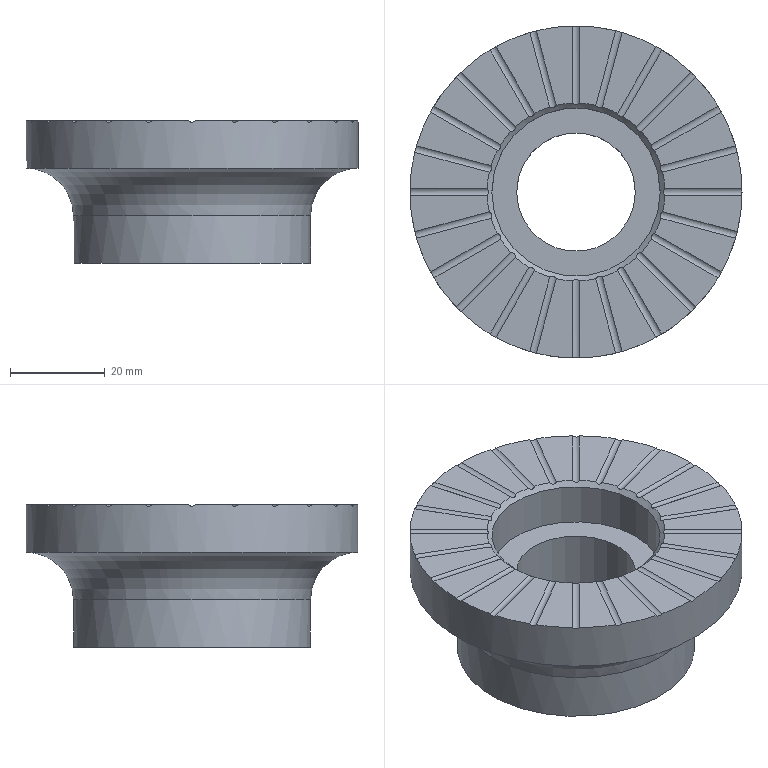Component | NX | TOP_PAD | 1 solid | 57 faces | volume 61498 mm3 | cylinder 28 | plane 26 | cone 2 | torus 1 | commonest cylinder face diameters 2 x24 50 x1 70 x1 25 x1 35.5 x1